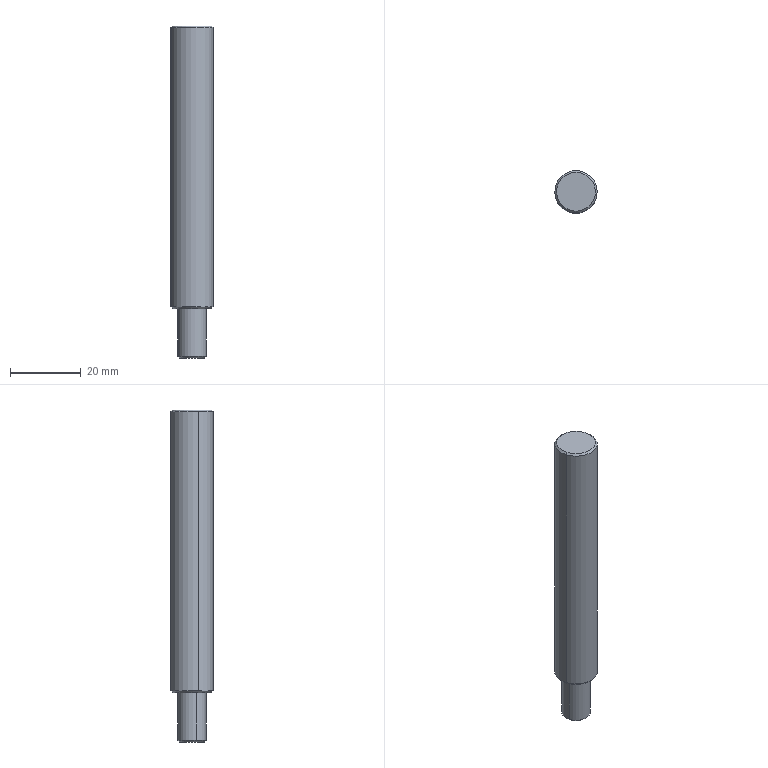Component | SolidWorks | DirectPressureVerticalSeal-1_GuidePost-2 | 1 solid | 13 faces | box 12 x 12 x 94 mm | volume 9739 mm3 | cone 6 | cylinder 4 | plane 3 | commonest cylinder face diameters 8 x2 12 x2
build123d program:
from build123d import *


with BuildPart() as part:
    # Sketch1 → Revolve1 (revolve)
    with BuildSketch(Plane.XY, mode=Mode.PRIVATE) as revolve1_sk:
        Polygon((0, 5.5), (0, 0), (94, 0), (94, 3.5), (93.5, 4), (80, 4), (80, 5.5), (79.5, 6), (0.5, 6), align=None)
    revolve(revolve1_sk.sketch.rotate(Axis((0, 0, 0), (1, 0, 0)), 270), axis=Axis((0, 0, 0), (1, 0, 0)))


solid = part.part

# Placed as in the assembly
solid = solid.moved(Location((-298.746, 181.873, 334.054), (0, 90, 0)))
STEP:
#1=COLOUR_RGB('',0.7922,0.8196,0.9333);
#2=FILL_AREA_STYLE_COLOUR('',#1);
#3=FILL_AREA_STYLE('',(#2));
#4=SURFACE_STYLE_FILL_AREA(#3);
#5=SURFACE_SIDE_STYLE('',(#4));
#6=SURFACE_STYLE_USAGE(.BOTH.,#5);
#7=PRESENTATION_STYLE_ASSIGNMENT((#6));
#8=CARTESIAN_POINT('',(-11.893,7.119,9.451));
#9=VERTEX_POINT('',#8);
#10=CARTESIAN_POINT('',(-11.63,7.201,9.451));
#11=VERTEX_POINT('',#10);
#12=CARTESIAN_POINT('',(-11.762,7.16,9.451));
#13=DIRECTION('',(0.,0.,-1.));
#14=DIRECTION('',(-0.9544,-0.2985,0.));
#15=AXIS2_PLACEMENT_3D('',#12,#13,#14);
#16=CIRCLE('',#15,0.1378);
#17=EDGE_CURVE('',#9,#11,#16,.T.);
#18=ORIENTED_EDGE('',*,*,#17,.F.);
#19=CARTESIAN_POINT('',(-11.912,7.113,9.471));
#20=VERTEX_POINT('',#19);
#21=CARTESIAN_POINT('',(-11.893,7.119,9.451));
#22=DIRECTION('',(-0.6749,-0.2111,0.7071));
#23=VECTOR('',#22,39.37);
#24=LINE('',#21,#23);
#25=EDGE_CURVE('',#9,#20,#24,.T.);
#26=ORIENTED_EDGE('',*,*,#25,.T.);
#27=CARTESIAN_POINT('',(-11.611,7.207,9.471));
#28=VERTEX_POINT('',#27);
#29=CARTESIAN_POINT('',(-11.762,7.16,9.471));
#30=DIRECTION('',(0.,0.,-1.));
#31=DIRECTION('',(-0.9544,-0.2985,0.));
#32=AXIS2_PLACEMENT_3D('',#29,#30,#31);
#33=CIRCLE('',#32,0.1575);
#34=EDGE_CURVE('',#20,#28,#33,.T.);
#35=ORIENTED_EDGE('',*,*,#34,.T.);
#36=CARTESIAN_POINT('',(-11.63,7.201,9.451));
#37=DIRECTION('',(0.6749,0.2111,0.7071));
#38=VECTOR('',#37,39.37);
#39=LINE('',#36,#38);
#40=EDGE_CURVE('',#11,#28,#39,.T.);
#41=ORIENTED_EDGE('',*,*,#40,.F.);
#42=EDGE_LOOP('',(#18,#26,#35,#41));
#43=FACE_OUTER_BOUND('',#42,.T.);
#44=CARTESIAN_POINT('',(-11.762,7.16,9.451));
#45=DIRECTION('',(-0.,-0.,1.));
#46=DIRECTION('',(0.9544,0.2985,0.));
#47=AXIS2_PLACEMENT_3D('',#44,#45,#46);
#48=CONICAL_SURFACE('',#47,0.1378,0.7854);
#49=ADVANCED_FACE('',(#43),#48,.T.);
#50=CARTESIAN_POINT('',(-11.912,7.113,10.002));
#51=VERTEX_POINT('',#50);
#52=CARTESIAN_POINT('',(-11.611,7.207,10.002));
#53=VERTEX_POINT('',#52);
#54=CARTESIAN_POINT('',(-11.762,7.16,10.002));
#55=DIRECTION('',(0.,0.,-1.));
#56=DIRECTION('',(-0.9544,-0.2985,0.));
#57=AXIS2_PLACEMENT_3D('',#54,#55,#56);
#58=CIRCLE('',#57,0.1575);
#59=EDGE_CURVE('',#51,#53,#58,.T.);
#60=ORIENTED_EDGE('',*,*,#59,.T.);
#61=CARTESIAN_POINT('',(-11.611,7.207,13.152));
#62=DIRECTION('',(0.,0.,-1.));
#63=VECTOR('',#62,39.37);
#64=LINE('',#61,#63);
#65=EDGE_CURVE('',#53,#28,#64,.T.);
#66=ORIENTED_EDGE('',*,*,#65,.T.);
#67=ORIENTED_EDGE('',*,*,#34,.F.);
#68=CARTESIAN_POINT('',(-11.912,7.113,13.152));
#69=DIRECTION('',(0.,0.,-1.));
#70=VECTOR('',#69,39.37);
#71=LINE('',#68,#70);
#72=EDGE_CURVE('',#51,#20,#71,.T.);
#73=ORIENTED_EDGE('',*,*,#72,.F.);
#74=EDGE_LOOP('',(#60,#66,#67,#73));
#75=FACE_OUTER_BOUND('',#74,.T.);
#76=CARTESIAN_POINT('',(-11.762,7.16,13.152));
#77=DIRECTION('',(0.,0.,-1.));
#78=DIRECTION('',(-0.9544,-0.2985,0.));
#79=AXIS2_PLACEMENT_3D('',#76,#77,#78);
#80=CYLINDRICAL_SURFACE('',#79,0.1575);
#81=ADVANCED_FACE('',(#75),#80,.T.);
#82=CARTESIAN_POINT('',(-11.968,7.096,10.002));
#83=VERTEX_POINT('',#82);
#84=CARTESIAN_POINT('',(-11.555,7.225,10.002));
#85=VERTEX_POINT('',#84);
#86=CARTESIAN_POINT('',(-11.762,7.16,10.002));
#87=DIRECTION('',(0.,0.,-1.));
#88=DIRECTION('',(-0.9544,-0.2985,0.));
#89=AXIS2_PLACEMENT_3D('',#86,#87,#88);
#90=CIRCLE('',#89,0.2165);
#91=EDGE_CURVE('',#83,#85,#90,.T.);
#92=ORIENTED_EDGE('',*,*,#91,.F.);
#93=CARTESIAN_POINT('',(-11.987,7.09,10.022));
#94=VERTEX_POINT('',#93);
#95=CARTESIAN_POINT('',(-11.968,7.096,10.002));
#96=DIRECTION('',(-0.6749,-0.2111,0.7071));
#97=VECTOR('',#96,39.37);
#98=LINE('',#95,#97);
#99=EDGE_CURVE('',#83,#94,#98,.T.);
#100=ORIENTED_EDGE('',*,*,#99,.T.);
#101=CARTESIAN_POINT('',(-11.536,7.231,10.022));
#102=VERTEX_POINT('',#101);
#103=CARTESIAN_POINT('',(-11.762,7.16,10.022));
#104=DIRECTION('',(0.,0.,-1.));
#105=DIRECTION('',(-0.9544,-0.2985,0.));
#106=AXIS2_PLACEMENT_3D('',#103,#104,#105);
#107=CIRCLE('',#106,0.2362);
#108=EDGE_CURVE('',#94,#102,#107,.T.);
#109=ORIENTED_EDGE('',*,*,#108,.T.);
#110=CARTESIAN_POINT('',(-11.555,7.225,10.002));
#111=DIRECTION('',(0.6749,0.2111,0.7071));
#112=VECTOR('',#111,39.37);
#113=LINE('',#110,#112);
#114=EDGE_CURVE('',#85,#102,#113,.T.);
#115=ORIENTED_EDGE('',*,*,#114,.F.);
#116=EDGE_LOOP('',(#92,#100,#109,#115));
#117=FACE_OUTER_BOUND('',#116,.T.);
#118=CARTESIAN_POINT('',(-11.762,7.16,10.002));
#119=DIRECTION('',(-0.,-0.,1.));
#120=DIRECTION('',(0.9544,0.2985,0.));
#121=AXIS2_PLACEMENT_3D('',#118,#119,#120);
#122=CONICAL_SURFACE('',#121,0.2165,0.7854);
#123=ADVANCED_FACE('',(#117),#122,.T.);
#124=CARTESIAN_POINT('',(-11.987,7.09,13.132));
#125=VERTEX_POINT('',#124);
#126=CARTESIAN_POINT('',(-11.536,7.231,13.132));
#127=VERTEX_POINT('',#126);
#128=CARTESIAN_POINT('',(-11.762,7.16,13.132));
#129=DIRECTION('',(0.,0.,-1.));
#130=DIRECTION('',(-0.9544,-0.2985,0.));
#131=AXIS2_PLACEMENT_3D('',#128,#129,#130);
#132=CIRCLE('',#131,0.2362);
#133=EDGE_CURVE('',#125,#127,#132,.T.);
#134=ORIENTED_EDGE('',*,*,#133,.T.);
#135=CARTESIAN_POINT('',(-11.536,7.231,13.152));
#136=DIRECTION('',(0.,0.,-1.));
#137=VECTOR('',#136,39.37);
#138=LINE('',#135,#137);
#139=EDGE_CURVE('',#127,#102,#138,.T.);
#140=ORIENTED_EDGE('',*,*,#139,.T.);
#141=ORIENTED_EDGE('',*,*,#108,.F.);
#142=CARTESIAN_POINT('',(-11.987,7.09,13.152));
#143=DIRECTION('',(0.,0.,-1.));
#144=VECTOR('',#143,39.37);
#145=LINE('',#142,#144);
#146=EDGE_CURVE('',#125,#94,#145,.T.);
#147=ORIENTED_EDGE('',*,*,#146,.F.);
#148=EDGE_LOOP('',(#134,#140,#141,#147));
#149=FACE_OUTER_BOUND('',#148,.T.);
#150=CARTESIAN_POINT('',(-11.762,7.16,13.152));
#151=DIRECTION('',(0.,0.,-1.));
#152=DIRECTION('',(-0.9544,-0.2985,0.));
#153=AXIS2_PLACEMENT_3D('',#150,#151,#152);
#154=CYLINDRICAL_SURFACE('',#153,0.2362);
#155=ADVANCED_FACE('',(#149),#154,.T.);
#156=CARTESIAN_POINT('',(-11.968,7.096,13.152));
#157=VERTEX_POINT('',#156);
#158=CARTESIAN_POINT('',(-11.555,7.225,13.152));
#159=VERTEX_POINT('',#158);
#160=CARTESIAN_POINT('',(-11.762,7.16,13.152));
#161=DIRECTION('',(0.,0.,-1.));
#162=DIRECTION('',(-0.9544,-0.2985,0.));
#163=AXIS2_PLACEMENT_3D('',#160,#161,#162);
#164=CIRCLE('',#163,0.2165);
#165=EDGE_CURVE('',#157,#159,#164,.T.);
#166=ORIENTED_EDGE('',*,*,#165,.T.);
#167=CARTESIAN_POINT('',(-11.536,7.231,13.132));
#168=DIRECTION('',(0.6749,0.2111,-0.7071));
#169=VECTOR('',#168,39.37);
#170=LINE('',#167,#169);
#171=EDGE_CURVE('',#159,#127,#170,.T.);
#172=ORIENTED_EDGE('',*,*,#171,.T.);
#173=ORIENTED_EDGE('',*,*,#133,.F.);
#174=CARTESIAN_POINT('',(-11.987,7.09,13.132));
#175=DIRECTION('',(-0.6749,-0.2111,-0.7071));
#176=VECTOR('',#175,39.37);
#177=LINE('',#174,#176);
#178=EDGE_CURVE('',#157,#125,#177,.T.);
#179=ORIENTED_EDGE('',*,*,#178,.F.);
#180=EDGE_LOOP('',(#166,#172,#173,#179));
#181=FACE_OUTER_BOUND('',#180,.T.);
#182=CARTESIAN_POINT('',(-11.762,7.16,13.132));
#183=DIRECTION('',(0.,0.,-1.));
#184=DIRECTION('',(-0.9544,-0.2985,0.));
#185=AXIS2_PLACEMENT_3D('',#182,#183,#184);
#186=CONICAL_SURFACE('',#185,0.2362,0.7854);
#187=ADVANCED_FACE('',(#181),#186,.T.);
#188=ORIENTED_EDGE('',*,*,#171,.F.);
#189=CARTESIAN_POINT('',(-11.762,7.16,13.152));
#190=DIRECTION('',(0.,0.,-1.));
#191=DIRECTION('',(-0.9544,-0.2985,0.));
#192=AXIS2_PLACEMENT_3D('',#189,#190,#191);
#193=CIRCLE('',#192,0.2165);
#194=EDGE_CURVE('',#159,#157,#193,.T.);
#195=ORIENTED_EDGE('',*,*,#194,.T.);
#196=ORIENTED_EDGE('',*,*,#178,.T.);
#197=CARTESIAN_POINT('',(-11.762,7.16,13.132));
#198=DIRECTION('',(0.,0.,-1.));
#199=DIRECTION('',(-0.9544,-0.2985,0.));
#200=AXIS2_PLACEMENT_3D('',#197,#198,#199);
#201=CIRCLE('',#200,0.2362);
#202=EDGE_CURVE('',#127,#125,#201,.T.);
#203=ORIENTED_EDGE('',*,*,#202,.F.);
#204=EDGE_LOOP('',(#188,#195,#196,#203));
#205=FACE_OUTER_BOUND('',#204,.T.);
#206=CARTESIAN_POINT('',(-11.762,7.16,13.132));
#207=DIRECTION('',(0.,0.,-1.));
#208=DIRECTION('',(-0.9544,-0.2985,0.));
#209=AXIS2_PLACEMENT_3D('',#206,#207,#208);
#210=CONICAL_SURFACE('',#209,0.2362,0.7854);
#211=ADVANCED_FACE('',(#205),#210,.T.);
#212=ORIENTED_EDGE('',*,*,#139,.F.);
#213=ORIENTED_EDGE('',*,*,#202,.T.);
#214=ORIENTED_EDGE('',*,*,#146,.T.);
#215=CARTESIAN_POINT('',(-11.762,7.16,10.022));
#216=DIRECTION('',(0.,0.,-1.));
#217=DIRECTION('',(-0.9544,-0.2985,0.));
#218=AXIS2_PLACEMENT_3D('',#215,#216,#217);
#219=CIRCLE('',#218,0.2362);
#220=EDGE_CURVE('',#102,#94,#219,.T.);
#221=ORIENTED_EDGE('',*,*,#220,.F.);
#222=EDGE_LOOP('',(#212,#213,#214,#221));
#223=FACE_OUTER_BOUND('',#222,.T.);
#224=CARTESIAN_POINT('',(-11.762,7.16,13.152));
#225=DIRECTION('',(0.,0.,-1.));
#226=DIRECTION('',(-0.9544,-0.2985,0.));
#227=AXIS2_PLACEMENT_3D('',#224,#225,#226);
#228=CYLINDRICAL_SURFACE('',#227,0.2362);
#229=ADVANCED_FACE('',(#223),#228,.T.);
#230=ORIENTED_EDGE('',*,*,#99,.F.);
#231=CARTESIAN_POINT('',(-11.762,7.16,10.002));
#232=DIRECTION('',(0.,0.,-1.));
#233=DIRECTION('',(-0.9544,-0.2985,0.));
#234=AXIS2_PLACEMENT_3D('',#231,#232,#233);
#235=CIRCLE('',#234,0.2165);
#236=EDGE_CURVE('',#85,#83,#235,.T.);
#237=ORIENTED_EDGE('',*,*,#236,.F.);
#238=ORIENTED_EDGE('',*,*,#114,.T.);
#239=ORIENTED_EDGE('',*,*,#220,.T.);
#240=EDGE_LOOP('',(#230,#237,#238,#239));
#241=FACE_OUTER_BOUND('',#240,.T.);
#242=CARTESIAN_POINT('',(-11.762,7.16,10.002));
#243=DIRECTION('',(-0.,-0.,1.));
#244=DIRECTION('',(0.9544,0.2985,0.));
#245=AXIS2_PLACEMENT_3D('',#242,#243,#244);
#246=CONICAL_SURFACE('',#245,0.2165,0.7854);
#247=ADVANCED_FACE('',(#241),#246,.T.);
#248=ORIENTED_EDGE('',*,*,#236,.T.);
#249=ORIENTED_EDGE('',*,*,#91,.T.);
#250=EDGE_LOOP('',(#248,#249));
#251=FACE_OUTER_BOUND('',#250,.T.);
#252=ORIENTED_EDGE('',*,*,#59,.F.);
#253=CARTESIAN_POINT('',(-11.762,7.16,10.002));
#254=DIRECTION('',(0.,0.,-1.));
#255=DIRECTION('',(-0.9544,-0.2985,0.));
#256=AXIS2_PLACEMENT_3D('',#253,#254,#255);
#257=CIRCLE('',#256,0.1575);
#258=EDGE_CURVE('',#53,#51,#257,.T.);
#259=ORIENTED_EDGE('',*,*,#258,.F.);
#260=EDGE_LOOP('',(#252,#259));
#261=FACE_BOUND('',#260,.T.);
#262=CARTESIAN_POINT('',(-11.809,7.311,10.002));
#263=DIRECTION('',(0.,0.,-1.));
#264=DIRECTION('',(-0.9544,-0.2985,-0.));
#265=AXIS2_PLACEMENT_3D('',#262,#263,#264);
#266=PLANE('',#265);
#267=ADVANCED_FACE('',(#251,#261),#266,.T.);
#268=ORIENTED_EDGE('',*,*,#65,.F.);
#269=ORIENTED_EDGE('',*,*,#258,.T.);
#270=ORIENTED_EDGE('',*,*,#72,.T.);
#271=CARTESIAN_POINT('',(-11.762,7.16,9.471));
#272=DIRECTION('',(0.,0.,-1.));
#273=DIRECTION('',(-0.9544,-0.2985,0.));
#274=AXIS2_PLACEMENT_3D('',#271,#272,#273);
#275=CIRCLE('',#274,0.1575);
#276=EDGE_CURVE('',#28,#20,#275,.T.);
#277=ORIENTED_EDGE('',*,*,#276,.F.);
#278=EDGE_LOOP('',(#268,#269,#270,#277));
#279=FACE_OUTER_BOUND('',#278,.T.);
#280=CARTESIAN_POINT('',(-11.762,7.16,13.152));
#281=DIRECTION('',(0.,0.,-1.));
#282=DIRECTION('',(-0.9544,-0.2985,0.));
#283=AXIS2_PLACEMENT_3D('',#280,#281,#282);
#284=CYLINDRICAL_SURFACE('',#283,0.1575);
#285=ADVANCED_FACE('',(#279),#284,.T.);
#286=ORIENTED_EDGE('',*,*,#25,.F.);
#287=CARTESIAN_POINT('',(-11.762,7.16,9.451));
#288=DIRECTION('',(0.,0.,-1.));
#289=DIRECTION('',(-0.9544,-0.2985,0.));
#290=AXIS2_PLACEMENT_3D('',#287,#288,#289);
#291=CIRCLE('',#290,0.1378);
#292=EDGE_CURVE('',#11,#9,#291,.T.);
#293=ORIENTED_EDGE('',*,*,#292,.F.);
#294=ORIENTED_EDGE('',*,*,#40,.T.);
#295=ORIENTED_EDGE('',*,*,#276,.T.);
#296=EDGE_LOOP('',(#286,#293,#294,#295));
#297=FACE_OUTER_BOUND('',#296,.T.);
#298=CARTESIAN_POINT('',(-11.762,7.16,9.451));
#299=DIRECTION('',(-0.,-0.,1.));
#300=DIRECTION('',(0.9544,0.2985,0.));
#301=AXIS2_PLACEMENT_3D('',#298,#299,#300);
#302=CONICAL_SURFACE('',#301,0.1378,0.7854);
#303=ADVANCED_FACE('',(#297),#302,.T.);
#304=ORIENTED_EDGE('',*,*,#292,.T.);
#305=ORIENTED_EDGE('',*,*,#17,.T.);
#306=EDGE_LOOP('',(#304,#305));
#307=FACE_OUTER_BOUND('',#306,.T.);
#308=CARTESIAN_POINT('',(-11.762,7.16,9.451));
#309=DIRECTION('',(0.,0.,-1.));
#310=DIRECTION('',(-0.9544,-0.2985,-0.));
#311=AXIS2_PLACEMENT_3D('',#308,#309,#310);
#312=PLANE('',#311);
#313=ADVANCED_FACE('',(#307),#312,.T.);
#314=ORIENTED_EDGE('',*,*,#165,.F.);
#315=ORIENTED_EDGE('',*,*,#194,.F.);
#316=EDGE_LOOP('',(#314,#315));
#317=FACE_OUTER_BOUND('',#316,.T.);
#318=CARTESIAN_POINT('',(-11.826,7.367,13.152));
#319=DIRECTION('',(-0.,-0.,1.));
#320=DIRECTION('',(0.9544,0.2985,0.));
#321=AXIS2_PLACEMENT_3D('',#318,#319,#320);
#322=PLANE('',#321);
#323=ADVANCED_FACE('',(#317),#322,.T.);
#324=CLOSED_SHELL('',(#49,#81,#123,#155,#187,#211,#229,#247,#267,#285,#303,#313,#323));
#325=MANIFOLD_SOLID_BREP('',#324);
#326=STYLED_ITEM('',(#7),#325);
#327=PRESENTATION_LAYER_ASSIGNMENT('','',(#326));
#328=(LENGTH_UNIT()NAMED_UNIT(*)SI_UNIT($,.METRE.));
#329=LENGTH_MEASURE_WITH_UNIT(LENGTH_MEASURE(0.0254),#328);
#330=DIMENSIONAL_EXPONENTS(1.,0.,0.,0.,0.,0.,0.);
#331=(CONVERSION_BASED_UNIT('',#329)LENGTH_UNIT()NAMED_UNIT(#330));
#332=UNCERTAINTY_MEASURE_WITH_UNIT(LENGTH_MEASURE(0.00001),#331,'','');
#333=(NAMED_UNIT(*)PLANE_ANGLE_UNIT()SI_UNIT($,.RADIAN.));
#334=(NAMED_UNIT(*)SI_UNIT($,.STERADIAN.)SOLID_ANGLE_UNIT());
#335=(GEOMETRIC_REPRESENTATION_CONTEXT(3)GLOBAL_UNCERTAINTY_ASSIGNED_CONTEXT((#332))GLOBAL_UNIT_ASSIGNED_CONTEXT((#331,#333,#334))REPRESENTATION_CONTEXT('',''));
#336=MECHANICAL_DESIGN_GEOMETRIC_PRESENTATION_REPRESENTATION('',(#326),#335);
#337=CARTESIAN_POINT('',(0.,0.,0.));
#338=DIRECTION('',(0.,0.,1.));
#339=DIRECTION('',(1.,0.,0.));
#340=AXIS2_PLACEMENT_3D('',#337,#338,#339);
#341=(LENGTH_UNIT()NAMED_UNIT(*)SI_UNIT($,.METRE.));
#342=LENGTH_MEASURE_WITH_UNIT(LENGTH_MEASURE(0.0254),#341);
#343=DIMENSIONAL_EXPONENTS(1.,0.,0.,0.,0.,0.,0.);
#344=(CONVERSION_BASED_UNIT('',#342)LENGTH_UNIT()NAMED_UNIT(#343));
#345=UNCERTAINTY_MEASURE_WITH_UNIT(LENGTH_MEASURE(0.00001),#344,'','');
#346=(NAMED_UNIT(*)PLANE_ANGLE_UNIT()SI_UNIT($,.RADIAN.));
#347=(NAMED_UNIT(*)SI_UNIT($,.STERADIAN.)SOLID_ANGLE_UNIT());
#348=(GEOMETRIC_REPRESENTATION_CONTEXT(3)GLOBAL_UNCERTAINTY_ASSIGNED_CONTEXT((#345))GLOBAL_UNIT_ASSIGNED_CONTEXT((#344,#346,#347))REPRESENTATION_CONTEXT('',''));
#349=ADVANCED_BREP_SHAPE_REPRESENTATION('',(#325,#340),#348);